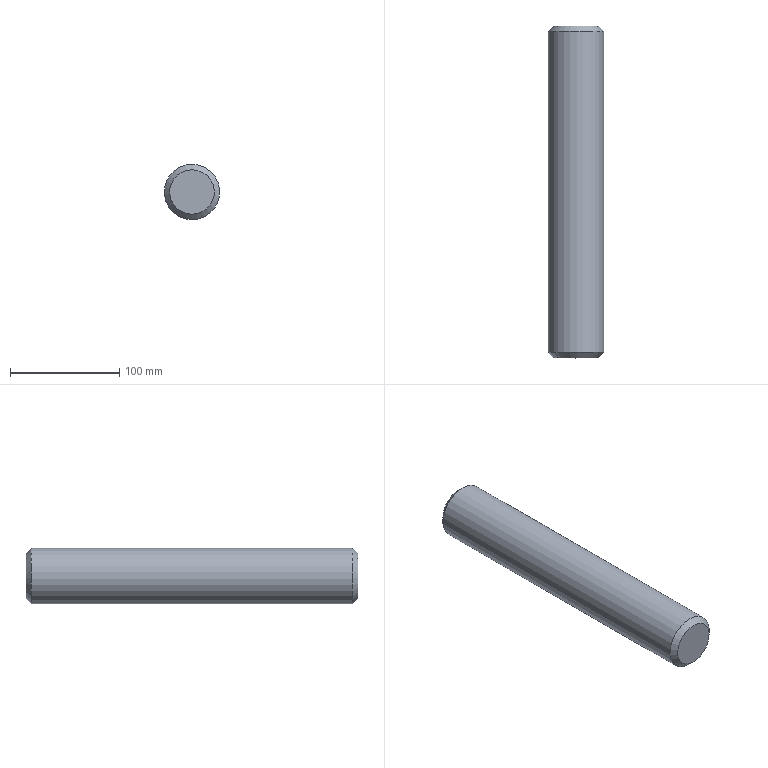Component | NX | PIN_304_4 | 1 solid | 5 faces | volume 612428 mm3 | plane 2 | cone 2 | cylinder 1 | commonest cylinder face diameters 50.8 x1